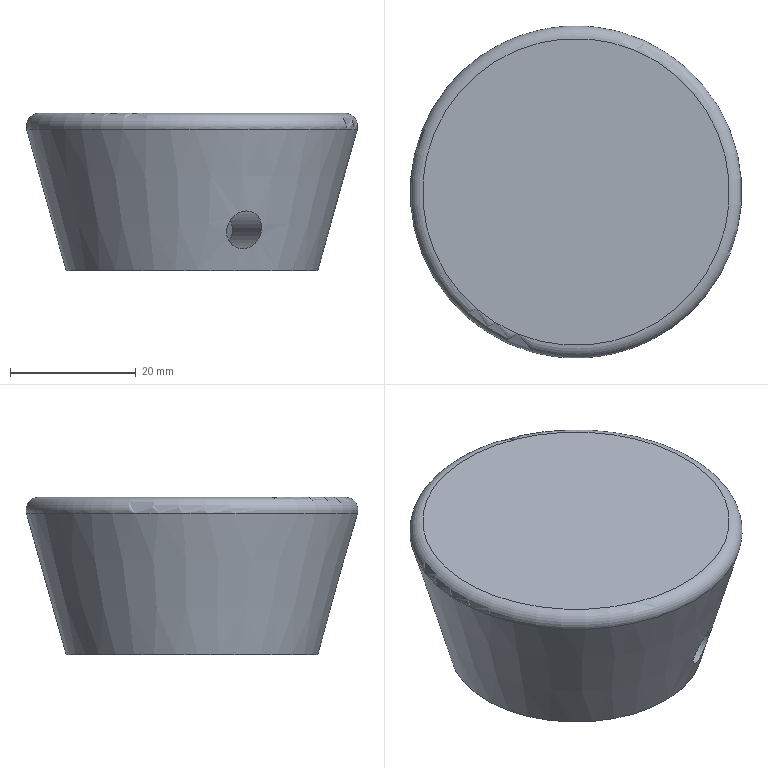Component | NX | TOPBLOCK | 1 solid | 7 faces | volume 37442 mm3 | plane 3 | cylinder 2 | cone 1 | torus 1 | commonest cylinder face diameters 20 x1 6 x1